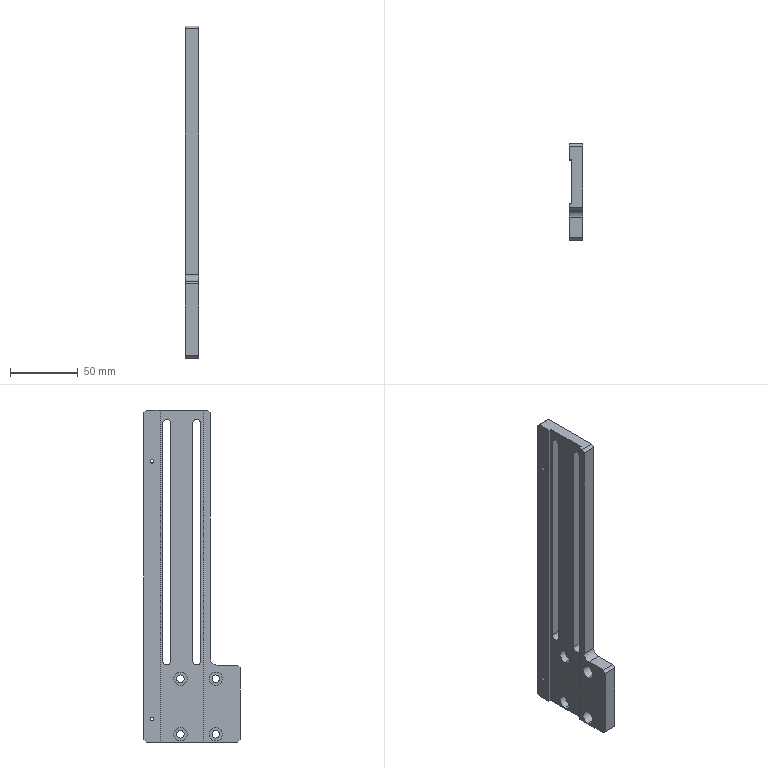Component | SolidWorks | MTCTV2104DJ006-000-0044SlidePlate2-2 | 1 solid | 68 faces | box 10 x 71 x 245 mm | volume 96553 mm3 | cylinder 35 | plane 25 | cone 8 | commonest cylinder face diameters 9.8 x8 5.5 x8 4.2 x8 6 x6 2.5 x4 10 x1
build123d program:
from build123d import *

# Parameters (mm, degrees)
SKETCH1_W                                           = 252
SKETCH1_H                                           = 71
BOSS_EXTRUDE1_DEPTH                                 = 10
SKETCH2_W                                           = 252
SKETCH2_H                                           = 32
CUT_EXTRUDE1_DEPTH                                  = 2
M5_TAPPED_HOLE1_D                                   = 4.2
M5_TAPPED_HOLE1_DEPTH                               = 14
M5_TAPPED_HOLE1_TIP                                 = 1.262
M3_TAPPED_HOLE1_D                                   = 2.5
CUT_EXTRUDE2_DEPTH                                  = 132.15
M5_TAPPED_HOLE2_D                                   = 4.2
M5_TAPPED_HOLE2_DEPTH                               = 14
M5_TAPPED_HOLE2_TIP                                 = 1.262
SKETCH10_W                                          = 204
SKETCH10_H                                          = 12
CUT_EXTRUDE3_DEPTH                                  = 132.287
FILLET1_R                                           = 5
CUT_EXTRUDE4_DEPTH                                  = 7
HOLE_SIZE_TYPE_OF_HEXAGON_SOCKET_HEAD_C_D           = 5.5
HOLE_SIZE_TYPE_OF_HEXAGON_SOCKET_HEAD_C_CBORE_D     = 9.8
HOLE_SIZE_TYPE_OF_HEXAGON_SOCKET_HEAD_C_CBORE_DEPTH = 7
LPATTERN1_COUNT                                     = 2
LPATTERN1_PITCH                                     = 41
SKETCH14_W                                          = 197
SKETCH14_H                                          = 12
BOSS_EXTRUDE2_DEPTH                                 = 10
SKETCH16_W                                          = 188.3
SKETCH16_H                                          = 22
CUT_EXTRUDE5_DEPTH                                  = 132.287
FILLET2_R                                           = 5
M3_TAPPED_HOLE2_D                                   = 2.5
CHAMFER1_SIZE                                       = 2


with BuildPart() as part:
    # Sketch1 → Boss-Extrude1 (new body)
    with BuildSketch(Plane.XY):
        Rectangle(SKETCH1_W, SKETCH1_H)
    extrude(amount=BOSS_EXTRUDE1_DEPTH)

    # Sketch2 → Cut-Extrude1 (cut)
    with BuildSketch(Plane.XY.offset(10)):
        with Locations((0, 7.5)):
            Rectangle(SKETCH2_W, SKETCH2_H)
    extrude(amount=-CUT_EXTRUDE1_DEPTH, mode=Mode.SUBTRACT)

    # M5 Tapped Hole1
    with Locations(Plane.ZY.offset(126)):
        with Locations((5, 30), (5, 0), (5, -30)):
            Hole(M5_TAPPED_HOLE1_D / 2, depth=M5_TAPPED_HOLE1_DEPTH)
            with Locations((0, 0, -(M5_TAPPED_HOLE1_DEPTH + M5_TAPPED_HOLE1_TIP / 2))):  # 118° drill point
                Cone(0, M5_TAPPED_HOLE1_D / 2, M5_TAPPED_HOLE1_TIP, mode=Mode.SUBTRACT)

    # M3 Tapped Hole1 (through all)
    with Locations(Plane.XY.offset(10)):
        with Locations((-109, 29.5), (81, 29.5)):
            Hole(M3_TAPPED_HOLE1_D / 2)

    # Sketch7 → Cut-Extrude2 (cut, through all)
    with BuildSketch(Plane.XY.offset(8)):
        with BuildLine():
            Line((-66, 21.5), (109, 21.5))
            ThreePointArc((109, 21.5), (112, 18.5), (109, 15.5))
            Line((109, 15.5), (-66, 15.5))
            ThreePointArc((-66, 15.5), (-69, 18.5), (-66, 21.5))
        make_face()
        with BuildLine():
            Line((-66, -0.5), (109, -0.5))
            ThreePointArc((109, -0.5), (112, -3.5), (109, -6.5))
            Line((109, -6.5), (-66, -6.5))
            ThreePointArc((-66, -6.5), (-69, -3.5), (-66, -0.5))
        make_face()
    extrude(amount=-CUT_EXTRUDE2_DEPTH, mode=Mode.SUBTRACT)

    # M5 Tapped Hole2
    with Locations(Plane(origin=(0, 35.5, 0), x_dir=(1, 0, 0), z_dir=(0, 1, 0))):
        with Locations((-86, -5)):
            Hole(M5_TAPPED_HOLE2_D / 2, depth=M5_TAPPED_HOLE2_DEPTH)
            with Locations((0, 0, -(M5_TAPPED_HOLE2_DEPTH + M5_TAPPED_HOLE2_TIP / 2))):  # 118° drill point
                Cone(0, M5_TAPPED_HOLE2_D / 2, M5_TAPPED_HOLE2_TIP, mode=Mode.SUBTRACT)

    # Sketch10 → Cut-Extrude3 (cut, through all)
    with BuildSketch(Plane.XY.offset(10)):
        with Locations((24, 29.5)):
            Rectangle(SKETCH10_W, SKETCH10_H)
    extrude(amount=-CUT_EXTRUDE3_DEPTH, mode=Mode.SUBTRACT)

    # Fillet1
    fillet1_edges = [part.edges().sort_by_distance(p)[0] for p in [
        (-78, 23.5, 4),
    ]]
    fillet(fillet1_edges, radius=FILLET1_R)

    # Sketch11 → Cut-Extrude4 (cut)
    with BuildSketch(Plane(origin=(126, 0, 0), x_dir=(0, 0, -1), z_dir=(1, 0, 0))):
        Polygon((0, -35.5), (0, 23.5), (-8, 23.5), (-8, -8.5), (-10, -8.5), (-10, -35.5), align=None)
    extrude(amount=-CUT_EXTRUDE4_DEPTH, mode=Mode.SUBTRACT)

    # Hole Size _Type of Hexagon Socket Head C (through all)
    with Locations(Plane.XY.offset(10)):
        with Locations((-120.3, 8.5), (-120.3, -17.5)):
            hole_size_type_of_hexagon_socket_head_c = CounterBoreHole(HOLE_SIZE_TYPE_OF_HEXAGON_SOCKET_HEAD_C_D / 2, HOLE_SIZE_TYPE_OF_HEXAGON_SOCKET_HEAD_C_CBORE_D / 2, HOLE_SIZE_TYPE_OF_HEXAGON_SOCKET_HEAD_C_CBORE_DEPTH)

    # LPattern1: Hole Size _Type of Hexagon Socket Head C ×2
    with Locations(*[(i * LPATTERN1_PITCH, 0, 0) for i in range(1, LPATTERN1_COUNT)]):
        add(hole_size_type_of_hexagon_socket_head_c, mode=Mode.SUBTRACT)

    # Sketch14 → Boss-Extrude2 (add)
    with BuildSketch(Plane.XY.offset(10)):
        with Locations((20.5, 29.5)):
            Rectangle(SKETCH14_W, SKETCH14_H)
    extrude(amount=-BOSS_EXTRUDE2_DEPTH)

    # Sketch16 → Cut-Extrude5 (cut, through all)
    with BuildSketch(Plane.XY.offset(10)):
        with Locations((24.85, -24.5)):
            Rectangle(SKETCH16_W, SKETCH16_H)
    extrude(amount=-CUT_EXTRUDE5_DEPTH, mode=Mode.SUBTRACT)

    # Fillet2
    fillet2_edges = [part.edges().sort_by_distance(p)[0] for p in [
        (-69.3, -13.5, 5),
    ]]
    fillet(fillet2_edges, radius=FILLET2_R)

    # M3 Tapped Hole2 (through all)
    with Locations(Plane.XY.offset(10)):
        with Locations((81, 29.5)):
            Hole(M3_TAPPED_HOLE2_D / 2)

    # Chamfer1
    chamfer1_edges = [part.edges().sort_by_distance(p)[0] for p in [
        (119, 35.5, 5),
        (119, -13.5, 5),
        (-69.3, -35.5, 5),
        (-126, -35.5, 5),
        (-126, 35.5, 5),
    ]]
    chamfer(chamfer1_edges, length=CHAMFER1_SIZE)


solid = part.part

# Placed as in the assembly
solid = solid.moved(Location((59.798, 22.281, 307.447), (0, -90, 0)))